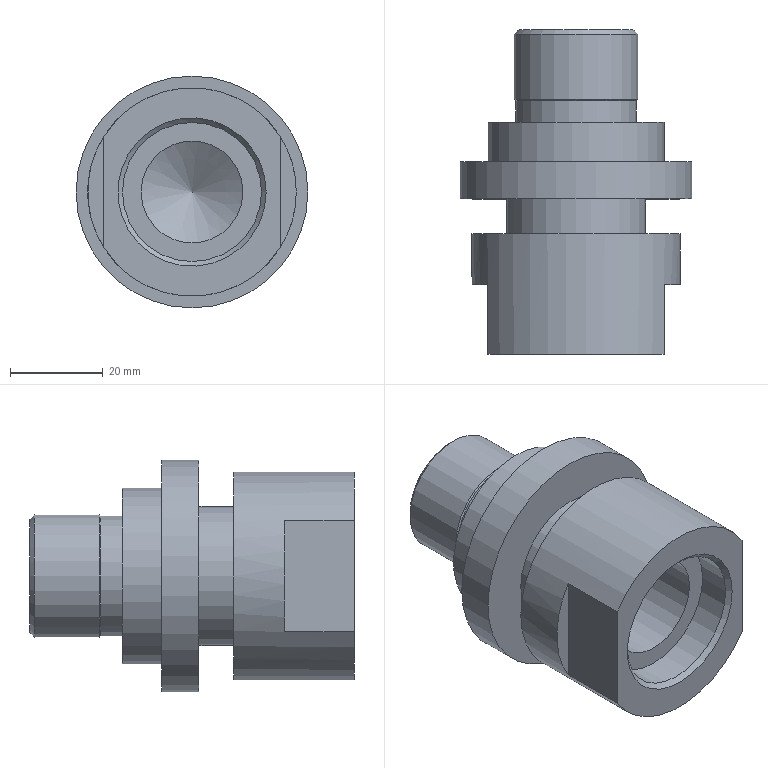Component | NX | PIVOT_SHAFT | 1 solid | 23 faces | volume 69022 mm3 | plane 11 | cylinder 8 | cone 4 | commonest cylinder face diameters 30 x2 45 x1 26.59 x1 26 x1 38 x1 50 x1 22 x1